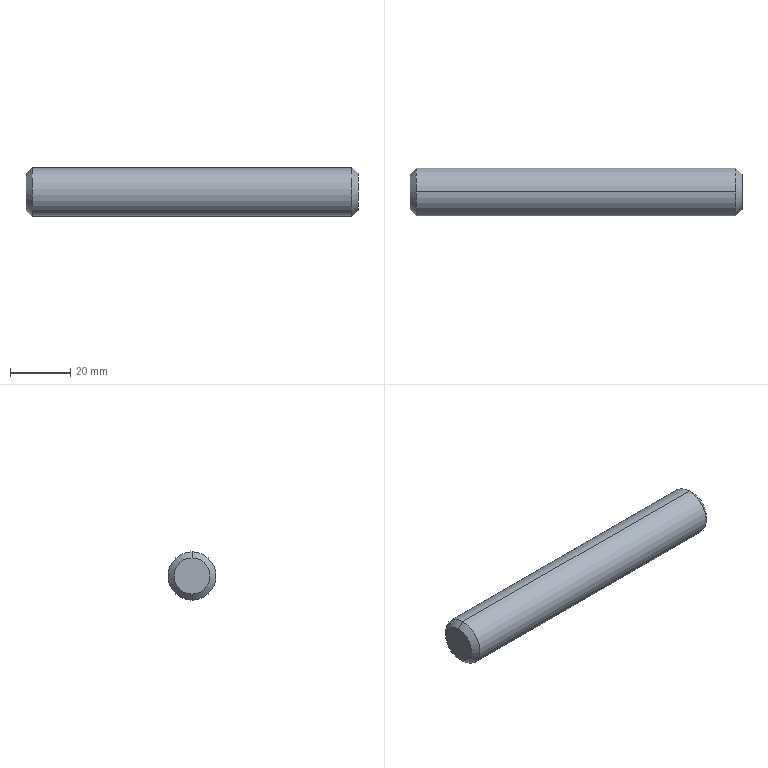Component | SolidWorks | Part4^CentrifugalDehydrator-2 | 1 solid | 8 faces | box 110 x 16 x 16 mm | volume 21933 mm3 | cone 4 | cylinder 2 | plane 2 | commonest cylinder face diameters 16 x2
STEP:
#1=COLOUR_RGB('',0.7922,0.8196,0.9333);
#2=FILL_AREA_STYLE_COLOUR('',#1);
#3=FILL_AREA_STYLE('',(#2));
#4=SURFACE_STYLE_FILL_AREA(#3);
#5=SURFACE_SIDE_STYLE('',(#4));
#6=SURFACE_STYLE_USAGE(.BOTH.,#5);
#7=PRESENTATION_STYLE_ASSIGNMENT((#6));
#8=CARTESIAN_POINT('',(-7.009,9.678,-2.986));
#9=VERTEX_POINT('',#8);
#10=CARTESIAN_POINT('',(-7.009,9.678,-3.458));
#11=VERTEX_POINT('',#10);
#12=CARTESIAN_POINT('',(-7.009,9.678,-3.222));
#13=DIRECTION('',(-1.,0.,0.));
#14=DIRECTION('',(0.,0.,1.));
#15=AXIS2_PLACEMENT_3D('',#12,#13,#14);
#16=CIRCLE('',#15,0.2362);
#17=EDGE_CURVE('',#9,#11,#16,.T.);
#18=ORIENTED_EDGE('',*,*,#17,.F.);
#19=CARTESIAN_POINT('',(-6.93,9.678,-2.907));
#20=VERTEX_POINT('',#19);
#21=CARTESIAN_POINT('',(-7.009,9.678,-2.986));
#22=DIRECTION('',(0.7071,0.,0.7071));
#23=VECTOR('',#22,39.37);
#24=LINE('',#21,#23);
#25=EDGE_CURVE('',#9,#20,#24,.T.);
#26=ORIENTED_EDGE('',*,*,#25,.T.);
#27=CARTESIAN_POINT('',(-6.93,9.678,-3.537));
#28=VERTEX_POINT('',#27);
#29=CARTESIAN_POINT('',(-6.93,9.678,-3.222));
#30=DIRECTION('',(1.,-0.,-0.));
#31=DIRECTION('',(0.,0.,1.));
#32=AXIS2_PLACEMENT_3D('',#29,#30,#31);
#33=CIRCLE('',#32,0.315);
#34=EDGE_CURVE('',#28,#20,#33,.T.);
#35=ORIENTED_EDGE('',*,*,#34,.F.);
#36=CARTESIAN_POINT('',(-7.009,9.678,-3.458));
#37=DIRECTION('',(0.7071,-0.,-0.7071));
#38=VECTOR('',#37,39.37);
#39=LINE('',#36,#38);
#40=EDGE_CURVE('',#11,#28,#39,.T.);
#41=ORIENTED_EDGE('',*,*,#40,.F.);
#42=EDGE_LOOP('',(#18,#26,#35,#41));
#43=FACE_OUTER_BOUND('',#42,.T.);
#44=CARTESIAN_POINT('',(-7.009,9.678,-3.222));
#45=DIRECTION('',(1.,-0.,-0.));
#46=DIRECTION('',(0.,0.,-1.));
#47=AXIS2_PLACEMENT_3D('',#44,#45,#46);
#48=CONICAL_SURFACE('',#47,0.2362,0.7854);
#49=ADVANCED_FACE('',(#43),#48,.T.);
#50=CARTESIAN_POINT('',(-2.678,9.678,-3.458));
#51=VERTEX_POINT('',#50);
#52=CARTESIAN_POINT('',(-2.678,9.678,-2.986));
#53=VERTEX_POINT('',#52);
#54=CARTESIAN_POINT('',(-2.678,9.678,-3.222));
#55=DIRECTION('',(1.,-0.,-0.));
#56=DIRECTION('',(0.,0.,1.));
#57=AXIS2_PLACEMENT_3D('',#54,#55,#56);
#58=CIRCLE('',#57,0.2362);
#59=EDGE_CURVE('',#51,#53,#58,.T.);
#60=ORIENTED_EDGE('',*,*,#59,.F.);
#61=CARTESIAN_POINT('',(-2.757,9.678,-3.537));
#62=VERTEX_POINT('',#61);
#63=CARTESIAN_POINT('',(-2.757,9.678,-3.537));
#64=DIRECTION('',(-0.7071,0.,-0.7071));
#65=VECTOR('',#64,39.37);
#66=LINE('',#63,#65);
#67=EDGE_CURVE('',#51,#62,#66,.T.);
#68=ORIENTED_EDGE('',*,*,#67,.T.);
#69=CARTESIAN_POINT('',(-2.757,9.678,-2.907));
#70=VERTEX_POINT('',#69);
#71=CARTESIAN_POINT('',(-2.757,9.678,-3.222));
#72=DIRECTION('',(-1.,0.,0.));
#73=DIRECTION('',(0.,0.,1.));
#74=AXIS2_PLACEMENT_3D('',#71,#72,#73);
#75=CIRCLE('',#74,0.315);
#76=EDGE_CURVE('',#70,#62,#75,.T.);
#77=ORIENTED_EDGE('',*,*,#76,.F.);
#78=CARTESIAN_POINT('',(-2.757,9.678,-2.907));
#79=DIRECTION('',(-0.7071,0.,0.7071));
#80=VECTOR('',#79,39.37);
#81=LINE('',#78,#80);
#82=EDGE_CURVE('',#53,#70,#81,.T.);
#83=ORIENTED_EDGE('',*,*,#82,.F.);
#84=EDGE_LOOP('',(#60,#68,#77,#83));
#85=FACE_OUTER_BOUND('',#84,.T.);
#86=CARTESIAN_POINT('',(-2.757,9.678,-3.222));
#87=DIRECTION('',(-1.,0.,0.));
#88=DIRECTION('',(0.,0.,1.));
#89=AXIS2_PLACEMENT_3D('',#86,#87,#88);
#90=CONICAL_SURFACE('',#89,0.315,0.7854);
#91=ADVANCED_FACE('',(#85),#90,.T.);
#92=ORIENTED_EDGE('',*,*,#76,.T.);
#93=CARTESIAN_POINT('',(-2.678,9.678,-3.537));
#94=DIRECTION('',(-1.,0.,0.));
#95=VECTOR('',#94,39.37);
#96=LINE('',#93,#95);
#97=EDGE_CURVE('',#62,#28,#96,.T.);
#98=ORIENTED_EDGE('',*,*,#97,.T.);
#99=ORIENTED_EDGE('',*,*,#34,.T.);
#100=CARTESIAN_POINT('',(-2.678,9.678,-2.907));
#101=DIRECTION('',(-1.,0.,0.));
#102=VECTOR('',#101,39.37);
#103=LINE('',#100,#102);
#104=EDGE_CURVE('',#70,#20,#103,.T.);
#105=ORIENTED_EDGE('',*,*,#104,.F.);
#106=EDGE_LOOP('',(#92,#98,#99,#105));
#107=FACE_OUTER_BOUND('',#106,.T.);
#108=CARTESIAN_POINT('',(-2.678,9.678,-3.222));
#109=DIRECTION('',(-1.,0.,0.));
#110=DIRECTION('',(0.,0.,1.));
#111=AXIS2_PLACEMENT_3D('',#108,#109,#110);
#112=CYLINDRICAL_SURFACE('',#111,0.315);
#113=ADVANCED_FACE('',(#107),#112,.T.);
#114=ORIENTED_EDGE('',*,*,#97,.F.);
#115=CARTESIAN_POINT('',(-2.757,9.678,-3.222));
#116=DIRECTION('',(-1.,0.,0.));
#117=DIRECTION('',(0.,0.,1.));
#118=AXIS2_PLACEMENT_3D('',#115,#116,#117);
#119=CIRCLE('',#118,0.315);
#120=EDGE_CURVE('',#62,#70,#119,.T.);
#121=ORIENTED_EDGE('',*,*,#120,.T.);
#122=ORIENTED_EDGE('',*,*,#104,.T.);
#123=CARTESIAN_POINT('',(-6.93,9.678,-3.222));
#124=DIRECTION('',(1.,-0.,-0.));
#125=DIRECTION('',(0.,0.,1.));
#126=AXIS2_PLACEMENT_3D('',#123,#124,#125);
#127=CIRCLE('',#126,0.315);
#128=EDGE_CURVE('',#20,#28,#127,.T.);
#129=ORIENTED_EDGE('',*,*,#128,.T.);
#130=EDGE_LOOP('',(#114,#121,#122,#129));
#131=FACE_OUTER_BOUND('',#130,.T.);
#132=CARTESIAN_POINT('',(-2.678,9.678,-3.222));
#133=DIRECTION('',(-1.,0.,0.));
#134=DIRECTION('',(0.,0.,1.));
#135=AXIS2_PLACEMENT_3D('',#132,#133,#134);
#136=CYLINDRICAL_SURFACE('',#135,0.315);
#137=ADVANCED_FACE('',(#131),#136,.T.);
#138=CARTESIAN_POINT('',(-2.678,9.678,-3.222));
#139=DIRECTION('',(1.,-0.,-0.));
#140=DIRECTION('',(0.,0.,1.));
#141=AXIS2_PLACEMENT_3D('',#138,#139,#140);
#142=CIRCLE('',#141,0.2362);
#143=EDGE_CURVE('',#53,#51,#142,.T.);
#144=ORIENTED_EDGE('',*,*,#143,.T.);
#145=ORIENTED_EDGE('',*,*,#59,.T.);
#146=EDGE_LOOP('',(#144,#145));
#147=FACE_OUTER_BOUND('',#146,.T.);
#148=CARTESIAN_POINT('',(-2.678,9.678,-3.222));
#149=DIRECTION('',(-1.,0.,0.));
#150=DIRECTION('',(0.,0.,1.));
#151=AXIS2_PLACEMENT_3D('',#148,#149,#150);
#152=PLANE('',#151);
#153=ADVANCED_FACE('',(#147),#152,.F.);
#154=CARTESIAN_POINT('',(-7.009,9.678,-3.222));
#155=DIRECTION('',(-1.,0.,0.));
#156=DIRECTION('',(0.,0.,1.));
#157=AXIS2_PLACEMENT_3D('',#154,#155,#156);
#158=CIRCLE('',#157,0.2362);
#159=EDGE_CURVE('',#11,#9,#158,.T.);
#160=ORIENTED_EDGE('',*,*,#159,.T.);
#161=ORIENTED_EDGE('',*,*,#17,.T.);
#162=EDGE_LOOP('',(#160,#161));
#163=FACE_OUTER_BOUND('',#162,.T.);
#164=CARTESIAN_POINT('',(-7.009,9.678,-3.222));
#165=DIRECTION('',(-1.,0.,0.));
#166=DIRECTION('',(0.,0.,1.));
#167=AXIS2_PLACEMENT_3D('',#164,#165,#166);
#168=PLANE('',#167);
#169=ADVANCED_FACE('',(#163),#168,.T.);
#170=ORIENTED_EDGE('',*,*,#67,.F.);
#171=ORIENTED_EDGE('',*,*,#143,.F.);
#172=ORIENTED_EDGE('',*,*,#82,.T.);
#173=ORIENTED_EDGE('',*,*,#120,.F.);
#174=EDGE_LOOP('',(#170,#171,#172,#173));
#175=FACE_OUTER_BOUND('',#174,.T.);
#176=CARTESIAN_POINT('',(-2.757,9.678,-3.222));
#177=DIRECTION('',(-1.,0.,0.));
#178=DIRECTION('',(0.,0.,1.));
#179=AXIS2_PLACEMENT_3D('',#176,#177,#178);
#180=CONICAL_SURFACE('',#179,0.315,0.7854);
#181=ADVANCED_FACE('',(#175),#180,.T.);
#182=ORIENTED_EDGE('',*,*,#25,.F.);
#183=ORIENTED_EDGE('',*,*,#159,.F.);
#184=ORIENTED_EDGE('',*,*,#40,.T.);
#185=ORIENTED_EDGE('',*,*,#128,.F.);
#186=EDGE_LOOP('',(#182,#183,#184,#185));
#187=FACE_OUTER_BOUND('',#186,.T.);
#188=CARTESIAN_POINT('',(-7.009,9.678,-3.222));
#189=DIRECTION('',(1.,-0.,-0.));
#190=DIRECTION('',(0.,0.,-1.));
#191=AXIS2_PLACEMENT_3D('',#188,#189,#190);
#192=CONICAL_SURFACE('',#191,0.2362,0.7854);
#193=ADVANCED_FACE('',(#187),#192,.T.);
#194=CLOSED_SHELL('',(#49,#91,#113,#137,#153,#169,#181,#193));
#195=MANIFOLD_SOLID_BREP('',#194);
#196=STYLED_ITEM('',(#7),#195);
#197=PRESENTATION_LAYER_ASSIGNMENT('','',(#196));
#198=CARTESIAN_POINT('',(0.,0.,0.));
#199=DIRECTION('',(0.,0.,1.));
#200=DIRECTION('',(1.,0.,0.));
#201=AXIS2_PLACEMENT_3D('',#198,#199,#200);
#202=(LENGTH_UNIT()NAMED_UNIT(*)SI_UNIT($,.METRE.));
#203=LENGTH_MEASURE_WITH_UNIT(LENGTH_MEASURE(0.0254),#202);
#204=DIMENSIONAL_EXPONENTS(1.,0.,0.,0.,0.,0.,0.);
#205=(CONVERSION_BASED_UNIT('',#203)LENGTH_UNIT()NAMED_UNIT(#204));
#206=UNCERTAINTY_MEASURE_WITH_UNIT(LENGTH_MEASURE(0.00001),#205,'','');
#207=(NAMED_UNIT(*)PLANE_ANGLE_UNIT()SI_UNIT($,.RADIAN.));
#208=(NAMED_UNIT(*)SI_UNIT($,.STERADIAN.)SOLID_ANGLE_UNIT());
#209=(GEOMETRIC_REPRESENTATION_CONTEXT(3)GLOBAL_UNCERTAINTY_ASSIGNED_CONTEXT((#206))GLOBAL_UNIT_ASSIGNED_CONTEXT((#205,#207,#208))REPRESENTATION_CONTEXT('',''));
#210=ADVANCED_BREP_SHAPE_REPRESENTATION('',(#195,#201),#209);
#211=(LENGTH_UNIT()NAMED_UNIT(*)SI_UNIT($,.METRE.));
#212=LENGTH_MEASURE_WITH_UNIT(LENGTH_MEASURE(0.0254),#211);
#213=DIMENSIONAL_EXPONENTS(1.,0.,0.,0.,0.,0.,0.);
#214=(CONVERSION_BASED_UNIT('',#212)LENGTH_UNIT()NAMED_UNIT(#213));
#215=UNCERTAINTY_MEASURE_WITH_UNIT(LENGTH_MEASURE(0.00001),#214,'','');
#216=(NAMED_UNIT(*)PLANE_ANGLE_UNIT()SI_UNIT($,.RADIAN.));
#217=(NAMED_UNIT(*)SI_UNIT($,.STERADIAN.)SOLID_ANGLE_UNIT());
#218=(GEOMETRIC_REPRESENTATION_CONTEXT(3)GLOBAL_UNCERTAINTY_ASSIGNED_CONTEXT((#215))GLOBAL_UNIT_ASSIGNED_CONTEXT((#214,#216,#217))REPRESENTATION_CONTEXT('',''));
#219=MECHANICAL_DESIGN_GEOMETRIC_PRESENTATION_REPRESENTATION('',(#196),#218);